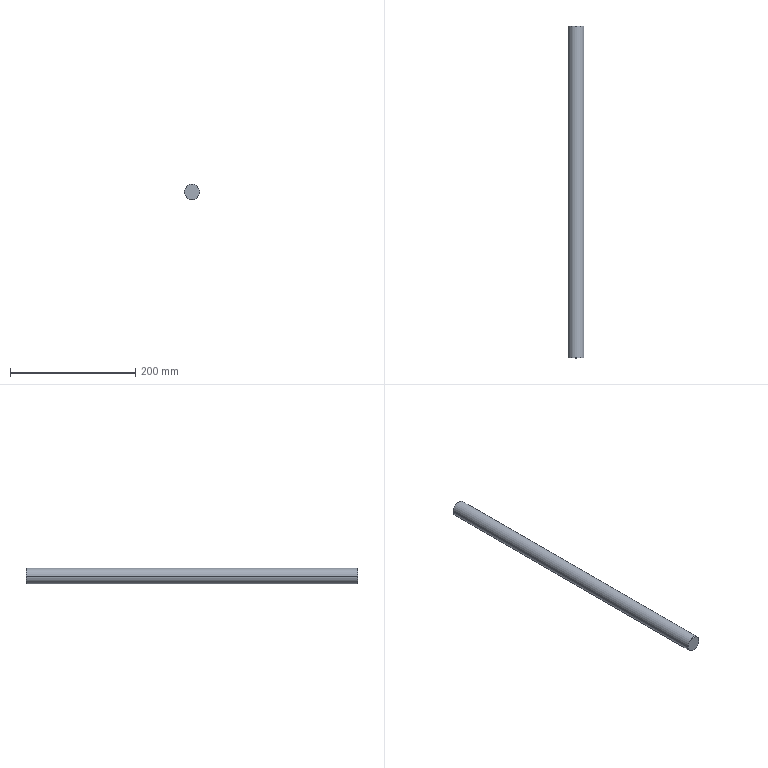Component | SolidWorks | CCDJSSupportColumn01-1 | 1 solid | 8 faces | box 25 x 530 x 25 mm | volume 260144 mm3 | cone 4 | cylinder 2 | plane 2 | commonest cylinder face diameters 25 x2
build123d program:
from build123d import *

# Parameters (mm, degrees)
SKETCH1_R           = 12.5
BOSS_EXTRUDE1_DEPTH = 530
CHAMFER1_SIZE       = 0.5


with BuildPart() as part:
    # Sketch1 → Boss-Extrude1 (new body)
    with BuildSketch(Plane.XY):
        Circle(SKETCH1_R)
    extrude(amount=BOSS_EXTRUDE1_DEPTH)

    # Chamfer1
    chamfer1_edges = [part.edges().sort_by_distance(p)[0] for p in [
        (-12.5, 0, 0),
        (-12.5, 0, 530),
    ]]
    chamfer(chamfer1_edges, length=CHAMFER1_SIZE)


solid = part.part

# Placed as in the assembly
solid = solid.moved(Location((30, 545, 0), (90, 0, 0)))
STEP:
#1=CARTESIAN_POINT('',(0.7087,21.457,0.));
#2=VERTEX_POINT('',#1);
#3=CARTESIAN_POINT('',(1.654,21.457,-0.));
#4=VERTEX_POINT('',#3);
#5=CARTESIAN_POINT('',(1.181,21.457,-0.));
#6=DIRECTION('',(0.,1.,0.));
#7=DIRECTION('',(1.,0.,0.));
#8=AXIS2_PLACEMENT_3D('',#5,#6,#7);
#9=CIRCLE('',#8,0.4724);
#10=EDGE_CURVE('',#2,#4,#9,.T.);
#11=ORIENTED_EDGE('',*,*,#10,.F.);
#12=CARTESIAN_POINT('',(0.689,21.437,-0.));
#13=VERTEX_POINT('',#12);
#14=CARTESIAN_POINT('',(0.689,21.437,0.));
#15=DIRECTION('',(-0.7071,-0.7071,0.));
#16=VECTOR('',#15,39.37);
#17=LINE('',#14,#16);
#18=EDGE_CURVE('',#2,#13,#17,.T.);
#19=ORIENTED_EDGE('',*,*,#18,.T.);
#20=CARTESIAN_POINT('',(1.673,21.437,0.));
#21=VERTEX_POINT('',#20);
#22=CARTESIAN_POINT('',(1.181,21.437,-0.));
#23=DIRECTION('',(0.,-1.,0.));
#24=DIRECTION('',(1.,0.,0.));
#25=AXIS2_PLACEMENT_3D('',#22,#23,#24);
#26=CIRCLE('',#25,0.4921);
#27=EDGE_CURVE('',#21,#13,#26,.T.);
#28=ORIENTED_EDGE('',*,*,#27,.F.);
#29=CARTESIAN_POINT('',(1.673,21.437,-0.));
#30=DIRECTION('',(0.7071,-0.7071,0.));
#31=VECTOR('',#30,39.37);
#32=LINE('',#29,#31);
#33=EDGE_CURVE('',#4,#21,#32,.T.);
#34=ORIENTED_EDGE('',*,*,#33,.F.);
#35=EDGE_LOOP('',(#11,#19,#28,#34));
#36=FACE_OUTER_BOUND('',#35,.T.);
#37=CARTESIAN_POINT('',(1.181,21.437,-0.));
#38=DIRECTION('',(0.,-1.,0.));
#39=DIRECTION('',(1.,0.,0.));
#40=AXIS2_PLACEMENT_3D('',#37,#38,#39);
#41=CONICAL_SURFACE('',#40,0.4921,0.7854);
#42=ADVANCED_FACE('',(#36),#41,.T.);
#43=CARTESIAN_POINT('',(1.654,0.5906,0.));
#44=VERTEX_POINT('',#43);
#45=CARTESIAN_POINT('',(0.7087,0.5906,-0.));
#46=VERTEX_POINT('',#45);
#47=CARTESIAN_POINT('',(1.181,0.5906,-0.));
#48=DIRECTION('',(0.,-1.,0.));
#49=DIRECTION('',(1.,0.,0.));
#50=AXIS2_PLACEMENT_3D('',#47,#48,#49);
#51=CIRCLE('',#50,0.4724);
#52=EDGE_CURVE('',#44,#46,#51,.T.);
#53=ORIENTED_EDGE('',*,*,#52,.F.);
#54=CARTESIAN_POINT('',(1.673,0.6102,0.));
#55=VERTEX_POINT('',#54);
#56=CARTESIAN_POINT('',(1.654,0.5906,0.));
#57=DIRECTION('',(0.7071,0.7071,0.));
#58=VECTOR('',#57,39.37);
#59=LINE('',#56,#58);
#60=EDGE_CURVE('',#44,#55,#59,.T.);
#61=ORIENTED_EDGE('',*,*,#60,.T.);
#62=CARTESIAN_POINT('',(0.689,0.6102,-0.));
#63=VERTEX_POINT('',#62);
#64=CARTESIAN_POINT('',(1.181,0.6102,-0.));
#65=DIRECTION('',(0.,1.,0.));
#66=DIRECTION('',(1.,0.,0.));
#67=AXIS2_PLACEMENT_3D('',#64,#65,#66);
#68=CIRCLE('',#67,0.4921);
#69=EDGE_CURVE('',#63,#55,#68,.T.);
#70=ORIENTED_EDGE('',*,*,#69,.F.);
#71=CARTESIAN_POINT('',(0.7087,0.5906,-0.));
#72=DIRECTION('',(-0.7071,0.7071,0.));
#73=VECTOR('',#72,39.37);
#74=LINE('',#71,#73);
#75=EDGE_CURVE('',#46,#63,#74,.T.);
#76=ORIENTED_EDGE('',*,*,#75,.F.);
#77=EDGE_LOOP('',(#53,#61,#70,#76));
#78=FACE_OUTER_BOUND('',#77,.T.);
#79=CARTESIAN_POINT('',(1.181,0.5906,-0.));
#80=DIRECTION('',(0.,1.,0.));
#81=DIRECTION('',(-1.,0.,0.));
#82=AXIS2_PLACEMENT_3D('',#79,#80,#81);
#83=CONICAL_SURFACE('',#82,0.4724,0.7854);
#84=ADVANCED_FACE('',(#78),#83,.T.);
#85=ORIENTED_EDGE('',*,*,#69,.T.);
#86=CARTESIAN_POINT('',(1.673,0.5906,0.));
#87=DIRECTION('',(0.,1.,0.));
#88=VECTOR('',#87,39.37);
#89=LINE('',#86,#88);
#90=EDGE_CURVE('',#55,#21,#89,.T.);
#91=ORIENTED_EDGE('',*,*,#90,.T.);
#92=ORIENTED_EDGE('',*,*,#27,.T.);
#93=CARTESIAN_POINT('',(0.689,0.5906,-0.));
#94=DIRECTION('',(0.,1.,0.));
#95=VECTOR('',#94,39.37);
#96=LINE('',#93,#95);
#97=EDGE_CURVE('',#63,#13,#96,.T.);
#98=ORIENTED_EDGE('',*,*,#97,.F.);
#99=EDGE_LOOP('',(#85,#91,#92,#98));
#100=FACE_OUTER_BOUND('',#99,.T.);
#101=CARTESIAN_POINT('',(1.181,0.5906,-0.));
#102=DIRECTION('',(0.,1.,0.));
#103=DIRECTION('',(-1.,0.,0.));
#104=AXIS2_PLACEMENT_3D('',#101,#102,#103);
#105=CYLINDRICAL_SURFACE('',#104,0.4921);
#106=ADVANCED_FACE('',(#100),#105,.T.);
#107=ORIENTED_EDGE('',*,*,#90,.F.);
#108=CARTESIAN_POINT('',(1.181,0.6102,-0.));
#109=DIRECTION('',(0.,1.,0.));
#110=DIRECTION('',(1.,0.,0.));
#111=AXIS2_PLACEMENT_3D('',#108,#109,#110);
#112=CIRCLE('',#111,0.4921);
#113=EDGE_CURVE('',#55,#63,#112,.T.);
#114=ORIENTED_EDGE('',*,*,#113,.T.);
#115=ORIENTED_EDGE('',*,*,#97,.T.);
#116=CARTESIAN_POINT('',(1.181,21.437,-0.));
#117=DIRECTION('',(0.,-1.,0.));
#118=DIRECTION('',(1.,0.,0.));
#119=AXIS2_PLACEMENT_3D('',#116,#117,#118);
#120=CIRCLE('',#119,0.4921);
#121=EDGE_CURVE('',#13,#21,#120,.T.);
#122=ORIENTED_EDGE('',*,*,#121,.T.);
#123=EDGE_LOOP('',(#107,#114,#115,#122));
#124=FACE_OUTER_BOUND('',#123,.T.);
#125=CARTESIAN_POINT('',(1.181,0.5906,-0.));
#126=DIRECTION('',(0.,1.,0.));
#127=DIRECTION('',(-1.,0.,0.));
#128=AXIS2_PLACEMENT_3D('',#125,#126,#127);
#129=CYLINDRICAL_SURFACE('',#128,0.4921);
#130=ADVANCED_FACE('',(#124),#129,.T.);
#131=CARTESIAN_POINT('',(1.181,0.5906,-0.));
#132=DIRECTION('',(0.,-1.,0.));
#133=DIRECTION('',(1.,0.,0.));
#134=AXIS2_PLACEMENT_3D('',#131,#132,#133);
#135=CIRCLE('',#134,0.4724);
#136=EDGE_CURVE('',#46,#44,#135,.T.);
#137=ORIENTED_EDGE('',*,*,#136,.T.);
#138=ORIENTED_EDGE('',*,*,#52,.T.);
#139=EDGE_LOOP('',(#137,#138));
#140=FACE_OUTER_BOUND('',#139,.T.);
#141=CARTESIAN_POINT('',(1.181,0.5906,-0.));
#142=DIRECTION('',(0.,-1.,0.));
#143=DIRECTION('',(1.,0.,0.));
#144=AXIS2_PLACEMENT_3D('',#141,#142,#143);
#145=PLANE('',#144);
#146=ADVANCED_FACE('',(#140),#145,.T.);
#147=CARTESIAN_POINT('',(1.181,21.457,-0.));
#148=DIRECTION('',(0.,1.,0.));
#149=DIRECTION('',(1.,0.,0.));
#150=AXIS2_PLACEMENT_3D('',#147,#148,#149);
#151=CIRCLE('',#150,0.4724);
#152=EDGE_CURVE('',#4,#2,#151,.T.);
#153=ORIENTED_EDGE('',*,*,#152,.T.);
#154=ORIENTED_EDGE('',*,*,#10,.T.);
#155=EDGE_LOOP('',(#153,#154));
#156=FACE_OUTER_BOUND('',#155,.T.);
#157=CARTESIAN_POINT('',(1.181,21.457,-0.));
#158=DIRECTION('',(0.,-1.,0.));
#159=DIRECTION('',(1.,0.,0.));
#160=AXIS2_PLACEMENT_3D('',#157,#158,#159);
#161=PLANE('',#160);
#162=ADVANCED_FACE('',(#156),#161,.F.);
#163=ORIENTED_EDGE('',*,*,#60,.F.);
#164=ORIENTED_EDGE('',*,*,#136,.F.);
#165=ORIENTED_EDGE('',*,*,#75,.T.);
#166=ORIENTED_EDGE('',*,*,#113,.F.);
#167=EDGE_LOOP('',(#163,#164,#165,#166));
#168=FACE_OUTER_BOUND('',#167,.T.);
#169=CARTESIAN_POINT('',(1.181,0.5906,-0.));
#170=DIRECTION('',(0.,1.,0.));
#171=DIRECTION('',(-1.,0.,0.));
#172=AXIS2_PLACEMENT_3D('',#169,#170,#171);
#173=CONICAL_SURFACE('',#172,0.4724,0.7854);
#174=ADVANCED_FACE('',(#168),#173,.T.);
#175=ORIENTED_EDGE('',*,*,#18,.F.);
#176=ORIENTED_EDGE('',*,*,#152,.F.);
#177=ORIENTED_EDGE('',*,*,#33,.T.);
#178=ORIENTED_EDGE('',*,*,#121,.F.);
#179=EDGE_LOOP('',(#175,#176,#177,#178));
#180=FACE_OUTER_BOUND('',#179,.T.);
#181=CARTESIAN_POINT('',(1.181,21.437,-0.));
#182=DIRECTION('',(0.,-1.,0.));
#183=DIRECTION('',(1.,0.,0.));
#184=AXIS2_PLACEMENT_3D('',#181,#182,#183);
#185=CONICAL_SURFACE('',#184,0.4921,0.7854);
#186=ADVANCED_FACE('',(#180),#185,.T.);
#187=CLOSED_SHELL('',(#42,#84,#106,#130,#146,#162,#174,#186));
#188=MANIFOLD_SOLID_BREP('',#187);
#189=CARTESIAN_POINT('',(0.,0.,0.));
#190=DIRECTION('',(0.,0.,1.));
#191=DIRECTION('',(1.,0.,0.));
#192=AXIS2_PLACEMENT_3D('',#189,#190,#191);
#193=(LENGTH_UNIT()NAMED_UNIT(*)SI_UNIT($,.METRE.));
#194=LENGTH_MEASURE_WITH_UNIT(LENGTH_MEASURE(0.0254),#193);
#195=DIMENSIONAL_EXPONENTS(1.,0.,0.,0.,0.,0.,0.);
#196=(CONVERSION_BASED_UNIT('',#194)LENGTH_UNIT()NAMED_UNIT(#195));
#197=UNCERTAINTY_MEASURE_WITH_UNIT(LENGTH_MEASURE(0.00001),#196,'','');
#198=(NAMED_UNIT(*)PLANE_ANGLE_UNIT()SI_UNIT($,.RADIAN.));
#199=(NAMED_UNIT(*)SI_UNIT($,.STERADIAN.)SOLID_ANGLE_UNIT());
#200=(GEOMETRIC_REPRESENTATION_CONTEXT(3)GLOBAL_UNCERTAINTY_ASSIGNED_CONTEXT((#197))GLOBAL_UNIT_ASSIGNED_CONTEXT((#196,#198,#199))REPRESENTATION_CONTEXT('',''));
#201=ADVANCED_BREP_SHAPE_REPRESENTATION('',(#188,#192),#200);
#202=COLOUR_RGB('',0.7922,0.8196,0.9333);
#203=FILL_AREA_STYLE_COLOUR('',#202);
#204=FILL_AREA_STYLE('',(#203));
#205=SURFACE_STYLE_FILL_AREA(#204);
#206=SURFACE_SIDE_STYLE('',(#205));
#207=SURFACE_STYLE_USAGE(.BOTH.,#206);
#208=PRESENTATION_STYLE_ASSIGNMENT((#207));
#209=STYLED_ITEM('',(#208),#188);
#210=PRESENTATION_LAYER_ASSIGNMENT('','',(#209));
#211=(LENGTH_UNIT()NAMED_UNIT(*)SI_UNIT($,.METRE.));
#212=LENGTH_MEASURE_WITH_UNIT(LENGTH_MEASURE(0.0254),#211);
#213=DIMENSIONAL_EXPONENTS(1.,0.,0.,0.,0.,0.,0.);
#214=(CONVERSION_BASED_UNIT('',#212)LENGTH_UNIT()NAMED_UNIT(#213));
#215=UNCERTAINTY_MEASURE_WITH_UNIT(LENGTH_MEASURE(0.00001),#214,'','');
#216=(NAMED_UNIT(*)PLANE_ANGLE_UNIT()SI_UNIT($,.RADIAN.));
#217=(NAMED_UNIT(*)SI_UNIT($,.STERADIAN.)SOLID_ANGLE_UNIT());
#218=(GEOMETRIC_REPRESENTATION_CONTEXT(3)GLOBAL_UNCERTAINTY_ASSIGNED_CONTEXT((#215))GLOBAL_UNIT_ASSIGNED_CONTEXT((#214,#216,#217))REPRESENTATION_CONTEXT('',''));
#219=MECHANICAL_DESIGN_GEOMETRIC_PRESENTATION_REPRESENTATION('',(#209),#218);